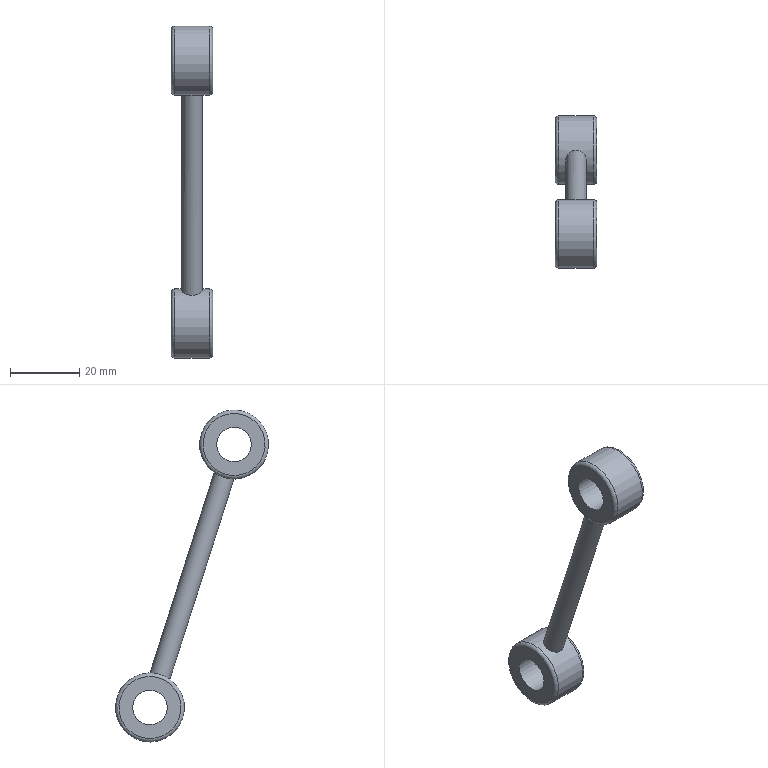Component | NX | CONNECTING_ROD | 1 solid | 13 faces | volume 7305 mm3 | cylinder 5 | plane 4 | torus 4 | commonest cylinder face diameters 10 x2 20 x2 6 x1